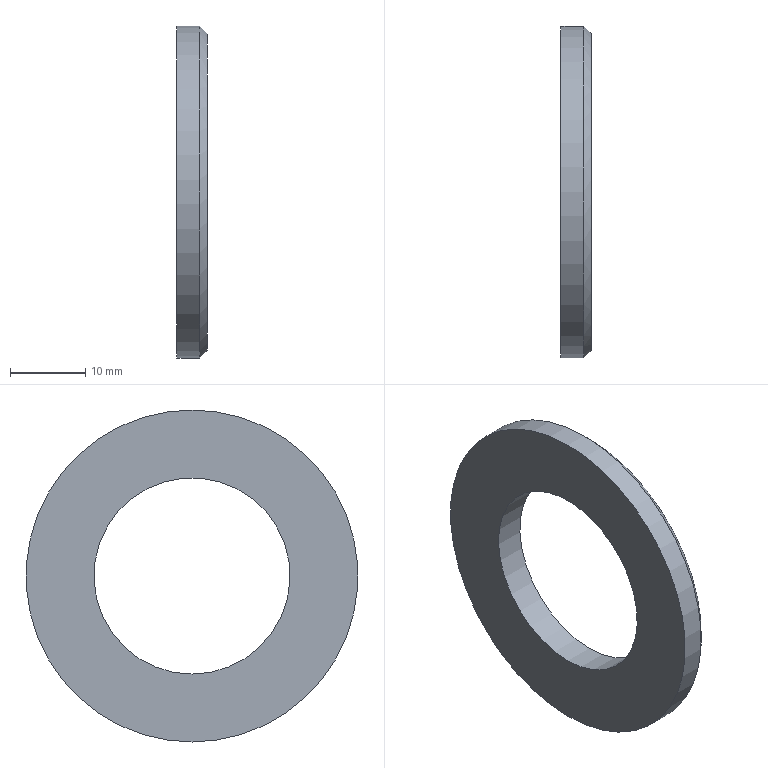Component | NX | 4_FLAT_WASHER | 1 solid | 5 faces | box 4 x 44 x 44 mm | volume 3890 mm3 | plane 2 | cylinder 2 | cone 1 | commonest cylinder face diameters 26 x1 44 x1
STEP:
#1=CARTESIAN_POINT('',(0.,0.,0.));
#2=DIRECTION('',(0.,0.,1.));
#3=DIRECTION('',(1.,0.,0.));
#4=AXIS2_PLACEMENT_3D('',#1,#2,#3);
#5=CARTESIAN_POINT('',(32.,0.,87.));
#6=VERTEX_POINT('',#5);
#7=CARTESIAN_POINT('',(32.,0.,100.));
#8=DIRECTION('',(-1.,0.,0.));
#9=DIRECTION('',(0.,0.,-1.));
#10=AXIS2_PLACEMENT_3D('',#7,#8,#9);
#11=CIRCLE('',#10,13.);
#12=CARTESIAN_POINT('',(32.,0.,122.));
#13=DIRECTION('',(1.,0.,0.));
#14=DIRECTION('',(0.,0.,1.));
#15=AXIS2_PLACEMENT_3D('',#12,#13,#14);
#16=PLANE('',#15);
#17=CARTESIAN_POINT('',(-35.,0.));
#18=CARTESIAN_POINT('',(-35.,22.517));
#19=CARTESIAN_POINT('',(-15.5,11.258));
#20=CARTESIAN_POINT('',(4.,0.));
#21=CARTESIAN_POINT('',(-15.5,-11.258));
#22=CARTESIAN_POINT('',(-35.,-22.517));
#23=CARTESIAN_POINT('',(-35.,0.));
#24=(BOUNDED_CURVE()B_SPLINE_CURVE(2,(#17,#18,#19,#20,#21,#22,#23),.UNSPECIFIED.,.T.,.F.)B_SPLINE_CURVE_WITH_KNOTS((1,2,2,2,2,1),(-2.094,0.,2.094,4.189,6.283,8.378),.UNSPECIFIED.)CURVE()GEOMETRIC_REPRESENTATION_ITEM()RATIONAL_B_SPLINE_CURVE((1.,0.5,1.,0.5,1.,0.5,1.))REPRESENTATION_ITEM(''));
#25=(GEOMETRIC_REPRESENTATION_CONTEXT(2)PARAMETRIC_REPRESENTATION_CONTEXT()REPRESENTATION_CONTEXT('',''));
#26=DEFINITIONAL_REPRESENTATION('',(#24),#25);
#27=PCURVE('',#16,#26);
#28=CARTESIAN_POINT('',(32.,0.,100.));
#29=DIRECTION('',(-1.,0.,0.));
#30=DIRECTION('',(0.,0.,-1.));
#31=AXIS2_PLACEMENT_3D('',#28,#29,#30);
#32=CYLINDRICAL_SURFACE('',#31,13.);
#33=CARTESIAN_POINT('',(0.,0.));
#34=DIRECTION('',(1.,0.));
#35=VECTOR('',#34,1.);
#36=LINE('',#33,#35);
#37=(GEOMETRIC_REPRESENTATION_CONTEXT(2)PARAMETRIC_REPRESENTATION_CONTEXT()REPRESENTATION_CONTEXT('',''));
#38=DEFINITIONAL_REPRESENTATION('',(#36),#37);
#39=PCURVE('',#32,#38);
#40=SURFACE_CURVE('',#11,(#27,#39),.PCURVE_S1.);
#41=EDGE_CURVE('',#6,#6,#40,.T.);
#42=ORIENTED_EDGE('',*,*,#41,.F.);
#43=EDGE_LOOP('',(#42));
#44=FACE_BOUND('',#43,.T.);
#45=CARTESIAN_POINT('',(32.,0.,78.));
#46=VERTEX_POINT('',#45);
#47=CARTESIAN_POINT('',(32.,0.,100.));
#48=DIRECTION('',(-1.,0.,0.));
#49=DIRECTION('',(0.,0.,-1.));
#50=AXIS2_PLACEMENT_3D('',#47,#48,#49);
#51=CIRCLE('',#50,22.);
#52=CARTESIAN_POINT('',(-44.,0.));
#53=CARTESIAN_POINT('',(-44.,38.105));
#54=CARTESIAN_POINT('',(-11.,19.053));
#55=CARTESIAN_POINT('',(22.,0.));
#56=CARTESIAN_POINT('',(-11.,-19.053));
#57=CARTESIAN_POINT('',(-44.,-38.105));
#58=CARTESIAN_POINT('',(-44.,0.));
#59=(BOUNDED_CURVE()B_SPLINE_CURVE(2,(#52,#53,#54,#55,#56,#57,#58),.UNSPECIFIED.,.T.,.F.)B_SPLINE_CURVE_WITH_KNOTS((1,2,2,2,2,1),(-2.094,0.,2.094,4.189,6.283,8.378),.UNSPECIFIED.)CURVE()GEOMETRIC_REPRESENTATION_ITEM()RATIONAL_B_SPLINE_CURVE((1.,0.5,1.,0.5,1.,0.5,1.))REPRESENTATION_ITEM(''));
#60=(GEOMETRIC_REPRESENTATION_CONTEXT(2)PARAMETRIC_REPRESENTATION_CONTEXT()REPRESENTATION_CONTEXT('',''));
#61=DEFINITIONAL_REPRESENTATION('',(#59),#60);
#62=PCURVE('',#16,#61);
#63=CARTESIAN_POINT('',(32.,0.,100.));
#64=DIRECTION('',(-1.,0.,0.));
#65=DIRECTION('',(0.,0.,-1.));
#66=AXIS2_PLACEMENT_3D('',#63,#64,#65);
#67=CYLINDRICAL_SURFACE('',#66,22.);
#68=CARTESIAN_POINT('',(0.,0.));
#69=DIRECTION('',(1.,0.));
#70=VECTOR('',#69,1.);
#71=LINE('',#68,#70);
#72=(GEOMETRIC_REPRESENTATION_CONTEXT(2)PARAMETRIC_REPRESENTATION_CONTEXT()REPRESENTATION_CONTEXT('',''));
#73=DEFINITIONAL_REPRESENTATION('',(#71),#72);
#74=PCURVE('',#67,#73);
#75=SURFACE_CURVE('',#51,(#62,#74),.PCURVE_S1.);
#76=EDGE_CURVE('',#46,#46,#75,.T.);
#77=ORIENTED_EDGE('',*,*,#76,.T.);
#78=EDGE_LOOP('',(#77));
#79=FACE_BOUND('',#78,.T.);
#80=ADVANCED_FACE('',(#44,#79),#16,.F.);
#81=CARTESIAN_POINT('',(36.,0.,87.));
#82=VERTEX_POINT('',#81);
#83=CARTESIAN_POINT('',(36.,0.,100.));
#84=DIRECTION('',(-1.,0.,0.));
#85=DIRECTION('',(0.,0.,-1.));
#86=AXIS2_PLACEMENT_3D('',#83,#84,#85);
#87=CIRCLE('',#86,13.);
#88=CARTESIAN_POINT('',(0.,-4.));
#89=DIRECTION('',(1.,0.));
#90=VECTOR('',#89,1.);
#91=LINE('',#88,#90);
#92=(GEOMETRIC_REPRESENTATION_CONTEXT(2)PARAMETRIC_REPRESENTATION_CONTEXT()REPRESENTATION_CONTEXT('',''));
#93=DEFINITIONAL_REPRESENTATION('',(#91),#92);
#94=PCURVE('',#32,#93);
#95=CARTESIAN_POINT('',(36.,0.,113.));
#96=DIRECTION('',(-1.,0.,0.));
#97=DIRECTION('',(0.,0.,-1.));
#98=AXIS2_PLACEMENT_3D('',#95,#96,#97);
#99=PLANE('',#98);
#100=CARTESIAN_POINT('',(13.,0.));
#101=DIRECTION('',(1.,0.));
#102=AXIS2_PLACEMENT_2D('',#100,#101);
#103=CIRCLE('',#102,13.);
#104=(GEOMETRIC_REPRESENTATION_CONTEXT(2)PARAMETRIC_REPRESENTATION_CONTEXT()REPRESENTATION_CONTEXT('',''));
#105=DEFINITIONAL_REPRESENTATION('',(#103),#104);
#106=PCURVE('',#99,#105);
#107=SURFACE_CURVE('',#87,(#94,#106),.PCURVE_S1.);
#108=EDGE_CURVE('',#82,#82,#107,.T.);
#109=ORIENTED_EDGE('',*,*,#108,.T.);
#110=CARTESIAN_POINT('',(36.,0.,87.));
#111=CARTESIAN_POINT('',(32.,0.,87.));
#112=B_SPLINE_CURVE_WITH_KNOTS('',1,(#110,#111),.UNSPECIFIED.,.F.,.F.,(2,2),(-4.,0.),.PIECEWISE_BEZIER_KNOTS.);
#113=CARTESIAN_POINT('',(6.283,0.));
#114=DIRECTION('',(0.,1.));
#115=VECTOR('',#114,1.);
#116=LINE('',#113,#115);
#117=(GEOMETRIC_REPRESENTATION_CONTEXT(2)PARAMETRIC_REPRESENTATION_CONTEXT()REPRESENTATION_CONTEXT('',''));
#118=DEFINITIONAL_REPRESENTATION('',(#116),#117);
#119=PCURVE('',#32,#118);
#120=CARTESIAN_POINT('',(0.,0.));
#121=DIRECTION('',(0.,1.));
#122=VECTOR('',#121,1.);
#123=LINE('',#120,#122);
#124=(GEOMETRIC_REPRESENTATION_CONTEXT(2)PARAMETRIC_REPRESENTATION_CONTEXT()REPRESENTATION_CONTEXT('',''));
#125=DEFINITIONAL_REPRESENTATION('',(#123),#124);
#126=PCURVE('',#32,#125);
#127=SEAM_CURVE('',#112,(#119,#126),.PCURVE_S1.);
#128=EDGE_CURVE('',#82,#6,#127,.T.);
#129=ORIENTED_EDGE('',*,*,#128,.T.);
#130=ORIENTED_EDGE('',*,*,#41,.F.);
#131=ORIENTED_EDGE('',*,*,#128,.F.);
#132=EDGE_LOOP('',(#109,#129,#130,#131));
#133=FACE_BOUND('',#132,.F.);
#134=ADVANCED_FACE('',(#133),#32,.F.);
#135=CARTESIAN_POINT('',(36.,0.,79.));
#136=VERTEX_POINT('',#135);
#137=CARTESIAN_POINT('',(36.,0.,100.));
#138=DIRECTION('',(1.,0.,0.));
#139=DIRECTION('',(0.,0.,-1.));
#140=AXIS2_PLACEMENT_3D('',#137,#138,#139);
#141=CIRCLE('',#140,21.);
#142=CARTESIAN_POINT('',(34.,0.));
#143=CARTESIAN_POINT('',(34.,-36.373));
#144=CARTESIAN_POINT('',(2.5,-18.187));
#145=CARTESIAN_POINT('',(-29.,-0.));
#146=CARTESIAN_POINT('',(2.5,18.187));
#147=CARTESIAN_POINT('',(34.,36.373));
#148=CARTESIAN_POINT('',(34.,0.));
#149=(BOUNDED_CURVE()B_SPLINE_CURVE(2,(#142,#143,#144,#145,#146,#147,#148),.UNSPECIFIED.,.T.,.F.)B_SPLINE_CURVE_WITH_KNOTS((1,2,2,2,2,1),(-2.094,0.,2.094,4.189,6.283,8.378),.UNSPECIFIED.)CURVE()GEOMETRIC_REPRESENTATION_ITEM()RATIONAL_B_SPLINE_CURVE((1.,0.5,1.,0.5,1.,0.5,1.))REPRESENTATION_ITEM(''));
#150=(GEOMETRIC_REPRESENTATION_CONTEXT(2)PARAMETRIC_REPRESENTATION_CONTEXT()REPRESENTATION_CONTEXT('',''));
#151=DEFINITIONAL_REPRESENTATION('',(#149),#150);
#152=PCURVE('',#99,#151);
#153=CARTESIAN_POINT('',(35.,0.,100.));
#154=DIRECTION('',(-1.,0.,0.));
#155=DIRECTION('',(0.,0.,-1.));
#156=AXIS2_PLACEMENT_3D('',#153,#154,#155);
#157=CONICAL_SURFACE('',#156,22.,0.7854);
#158=CARTESIAN_POINT('',(6.283,-1.));
#159=DIRECTION('',(-1.,0.));
#160=VECTOR('',#159,1.);
#161=LINE('',#158,#160);
#162=(GEOMETRIC_REPRESENTATION_CONTEXT(2)PARAMETRIC_REPRESENTATION_CONTEXT()REPRESENTATION_CONTEXT('',''));
#163=DEFINITIONAL_REPRESENTATION('',(#161),#162);
#164=PCURVE('',#157,#163);
#165=SURFACE_CURVE('',#141,(#152,#164),.PCURVE_S1.);
#166=EDGE_CURVE('',#136,#136,#165,.T.);
#167=ORIENTED_EDGE('',*,*,#166,.T.);
#168=EDGE_LOOP('',(#167));
#169=FACE_BOUND('',#168,.T.);
#170=ORIENTED_EDGE('',*,*,#108,.T.);
#171=EDGE_LOOP('',(#170));
#172=FACE_BOUND('',#171,.T.);
#173=ADVANCED_FACE('',(#169,#172),#99,.F.);
#174=CARTESIAN_POINT('',(35.,0.,78.));
#175=VERTEX_POINT('',#174);
#176=CARTESIAN_POINT('',(35.,0.,100.));
#177=DIRECTION('',(-1.,0.,0.));
#178=DIRECTION('',(0.,0.,-1.));
#179=AXIS2_PLACEMENT_3D('',#176,#177,#178);
#180=CIRCLE('',#179,22.);
#181=CARTESIAN_POINT('',(0.,-3.));
#182=DIRECTION('',(1.,0.));
#183=VECTOR('',#182,1.);
#184=LINE('',#181,#183);
#185=(GEOMETRIC_REPRESENTATION_CONTEXT(2)PARAMETRIC_REPRESENTATION_CONTEXT()REPRESENTATION_CONTEXT('',''));
#186=DEFINITIONAL_REPRESENTATION('',(#184),#185);
#187=PCURVE('',#67,#186);
#188=CARTESIAN_POINT('',(0.,0.));
#189=DIRECTION('',(1.,0.));
#190=VECTOR('',#189,1.);
#191=LINE('',#188,#190);
#192=(GEOMETRIC_REPRESENTATION_CONTEXT(2)PARAMETRIC_REPRESENTATION_CONTEXT()REPRESENTATION_CONTEXT('',''));
#193=DEFINITIONAL_REPRESENTATION('',(#191),#192);
#194=PCURVE('',#157,#193);
#195=SURFACE_CURVE('',#180,(#187,#194),.PCURVE_S1.);
#196=EDGE_CURVE('',#175,#175,#195,.T.);
#197=ORIENTED_EDGE('',*,*,#196,.T.);
#198=CARTESIAN_POINT('',(35.,0.,78.));
#199=CARTESIAN_POINT('',(32.,0.,78.));
#200=B_SPLINE_CURVE_WITH_KNOTS('',1,(#198,#199),.UNSPECIFIED.,.F.,.F.,(2,2),(-3.,0.),.PIECEWISE_BEZIER_KNOTS.);
#201=CARTESIAN_POINT('',(6.283,0.));
#202=DIRECTION('',(0.,1.));
#203=VECTOR('',#202,1.);
#204=LINE('',#201,#203);
#205=(GEOMETRIC_REPRESENTATION_CONTEXT(2)PARAMETRIC_REPRESENTATION_CONTEXT()REPRESENTATION_CONTEXT('',''));
#206=DEFINITIONAL_REPRESENTATION('',(#204),#205);
#207=PCURVE('',#67,#206);
#208=CARTESIAN_POINT('',(0.,0.));
#209=DIRECTION('',(0.,1.));
#210=VECTOR('',#209,1.);
#211=LINE('',#208,#210);
#212=(GEOMETRIC_REPRESENTATION_CONTEXT(2)PARAMETRIC_REPRESENTATION_CONTEXT()REPRESENTATION_CONTEXT('',''));
#213=DEFINITIONAL_REPRESENTATION('',(#211),#212);
#214=PCURVE('',#67,#213);
#215=SEAM_CURVE('',#200,(#207,#214),.PCURVE_S1.);
#216=EDGE_CURVE('',#175,#46,#215,.T.);
#217=ORIENTED_EDGE('',*,*,#216,.T.);
#218=ORIENTED_EDGE('',*,*,#76,.F.);
#219=ORIENTED_EDGE('',*,*,#216,.F.);
#220=EDGE_LOOP('',(#197,#217,#218,#219));
#221=FACE_BOUND('',#220,.T.);
#222=ADVANCED_FACE('',(#221),#67,.T.);
#223=ORIENTED_EDGE('',*,*,#166,.F.);
#224=CARTESIAN_POINT('',(36.,0.,79.));
#225=CARTESIAN_POINT('',(35.,0.,78.));
#226=B_SPLINE_CURVE_WITH_KNOTS('',1,(#224,#225),.UNSPECIFIED.,.F.,.F.,(2,2),(-1.414,0.),.PIECEWISE_BEZIER_KNOTS.);
#227=CARTESIAN_POINT('',(6.283,0.));
#228=DIRECTION('',(0.,1.));
#229=VECTOR('',#228,1.);
#230=LINE('',#227,#229);
#231=(GEOMETRIC_REPRESENTATION_CONTEXT(2)PARAMETRIC_REPRESENTATION_CONTEXT()REPRESENTATION_CONTEXT('',''));
#232=DEFINITIONAL_REPRESENTATION('',(#230),#231);
#233=PCURVE('',#157,#232);
#234=CARTESIAN_POINT('',(0.,0.));
#235=DIRECTION('',(0.,1.));
#236=VECTOR('',#235,1.);
#237=LINE('',#234,#236);
#238=(GEOMETRIC_REPRESENTATION_CONTEXT(2)PARAMETRIC_REPRESENTATION_CONTEXT()REPRESENTATION_CONTEXT('',''));
#239=DEFINITIONAL_REPRESENTATION('',(#237),#238);
#240=PCURVE('',#157,#239);
#241=SEAM_CURVE('',#226,(#233,#240),.PCURVE_S1.);
#242=EDGE_CURVE('',#136,#175,#241,.T.);
#243=ORIENTED_EDGE('',*,*,#242,.T.);
#244=ORIENTED_EDGE('',*,*,#196,.F.);
#245=ORIENTED_EDGE('',*,*,#242,.F.);
#246=EDGE_LOOP('',(#223,#243,#244,#245));
#247=FACE_BOUND('',#246,.T.);
#248=ADVANCED_FACE('',(#247),#157,.T.);
#249=CLOSED_SHELL('',(#80,#134,#173,#222,#248));
#250=MANIFOLD_SOLID_BREP('',#249);
#251=(LENGTH_UNIT()NAMED_UNIT(*)SI_UNIT(.MILLI.,.METRE.));
#252=UNCERTAINTY_MEASURE_WITH_UNIT(LENGTH_MEASURE(0.00001),#251,'','');
#253=(NAMED_UNIT(*)PLANE_ANGLE_UNIT()SI_UNIT($,.RADIAN.));
#254=(NAMED_UNIT(*)SI_UNIT($,.STERADIAN.)SOLID_ANGLE_UNIT());
#255=(GEOMETRIC_REPRESENTATION_CONTEXT(3)GLOBAL_UNCERTAINTY_ASSIGNED_CONTEXT((#252))GLOBAL_UNIT_ASSIGNED_CONTEXT((#251,#253,#254))REPRESENTATION_CONTEXT('',''));
#256=ADVANCED_BREP_SHAPE_REPRESENTATION('',(#4,#250),#255);